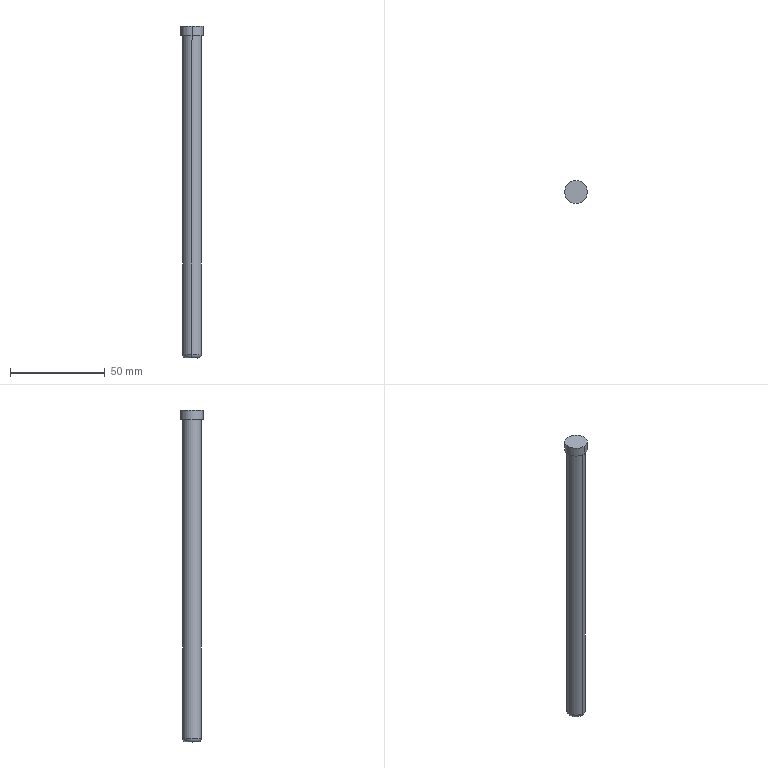Component | SolidWorks | 2SZT-2-003-5 | 1 solid | 9 faces | box 12 x 12 x 175 mm | volume 13893 mm3 | cylinder 4 | plane 3 | torus 2 | commonest cylinder face diameters 12 x2 10 x2
build123d program:
from build123d import *

# Parameters (mm, degrees)
SKETCH1_R           = 5
BOSS_EXTRUDE1_DEPTH = 170
SKETCH2_R           = 6
BOSS_EXTRUDE2_DEPTH = 5
FILLET1_R           = 2


with BuildPart() as part:
    # Sketch1 → Boss-Extrude1 (new body)
    with BuildSketch(Plane(origin=(0, 0, 0), x_dir=(1, 0, 0), z_dir=(0, 1, 0))):
        with Locations(Location((0, 0, 0), (0, 0, 270))):
            Circle(SKETCH1_R)
    extrude(amount=BOSS_EXTRUDE1_DEPTH)

    # Sketch2 → Boss-Extrude2 (add)
    with BuildSketch(Plane.XZ):
        with Locations(Location((0, 0, 0), (0, 0, 270))):
            Circle(SKETCH2_R)
    extrude(amount=BOSS_EXTRUDE2_DEPTH)

    # Fillet1
    fillet1_edges = [part.edges().sort_by_distance(p)[0] for p in [
        (0, 170, -5),
    ]]
    fillet(fillet1_edges, radius=FILLET1_R)


solid = part.part

# Placed as in the assembly
solid = solid.moved(Location((1050.266, 384.385, -180.948), (-90, 0, 0)))
STEP:
#1=COLOUR_RGB('',0.7922,0.8196,0.9333);
#2=FILL_AREA_STYLE_COLOUR('',#1);
#3=FILL_AREA_STYLE('',(#2));
#4=SURFACE_STYLE_FILL_AREA(#3);
#5=SURFACE_SIDE_STYLE('',(#4));
#6=SURFACE_STYLE_USAGE(.BOTH.,#5);
#7=PRESENTATION_STYLE_ASSIGNMENT((#6));
#8=CARTESIAN_POINT('',(41.349,14.936,-13.738));
#9=VERTEX_POINT('',#8);
#10=CARTESIAN_POINT('',(41.349,15.33,-13.738));
#11=VERTEX_POINT('',#10);
#12=CARTESIAN_POINT('',(41.349,15.133,-13.738));
#13=DIRECTION('',(0.00002551,0.,1.));
#14=DIRECTION('',(-0.00002551,1.,0.));
#15=AXIS2_PLACEMENT_3D('',#12,#13,#14);
#16=CIRCLE('',#15,0.1969);
#17=EDGE_CURVE('',#9,#11,#16,.T.);
#18=ORIENTED_EDGE('',*,*,#17,.F.);
#19=CARTESIAN_POINT('',(41.349,15.015,-13.817));
#20=VERTEX_POINT('',#19);
#21=CARTESIAN_POINT('',(41.349,15.015,-13.738));
#22=DIRECTION('',(1.,0.00002551,-0.00002551));
#23=DIRECTION('',(-0.00002551,1.,0.));
#24=AXIS2_PLACEMENT_3D('',#21,#22,#23);
#25=CIRCLE('',#24,0.07874);
#26=EDGE_CURVE('',#9,#20,#25,.T.);
#27=ORIENTED_EDGE('',*,*,#26,.T.);
#28=CARTESIAN_POINT('',(41.349,15.251,-13.817));
#29=VERTEX_POINT('',#28);
#30=CARTESIAN_POINT('',(41.349,15.133,-13.817));
#31=DIRECTION('',(-0.00002551,-0.,-1.));
#32=DIRECTION('',(-0.00002551,1.,0.));
#33=AXIS2_PLACEMENT_3D('',#30,#31,#32);
#34=CIRCLE('',#33,0.1181);
#35=EDGE_CURVE('',#29,#20,#34,.T.);
#36=ORIENTED_EDGE('',*,*,#35,.F.);
#37=CARTESIAN_POINT('',(41.349,15.251,-13.738));
#38=DIRECTION('',(-1.,-0.00002551,0.00002551));
#39=DIRECTION('',(0.00002551,-1.,0.));
#40=AXIS2_PLACEMENT_3D('',#37,#38,#39);
#41=CIRCLE('',#40,0.07874);
#42=EDGE_CURVE('',#11,#29,#41,.T.);
#43=ORIENTED_EDGE('',*,*,#42,.F.);
#44=EDGE_LOOP('',(#18,#27,#36,#43));
#45=FACE_OUTER_BOUND('',#44,.T.);
#46=CARTESIAN_POINT('',(41.349,15.133,-13.738));
#47=DIRECTION('',(-0.00002551,-0.,-1.));
#48=DIRECTION('',(-0.00002551,1.,0.));
#49=AXIS2_PLACEMENT_3D('',#46,#47,#48);
#50=TOROIDAL_SURFACE('',#49,0.1181,0.07874);
#51=ADVANCED_FACE('',(#45),#50,.T.);
#52=CARTESIAN_POINT('',(41.349,14.897,-6.927));
#53=VERTEX_POINT('',#52);
#54=CARTESIAN_POINT('',(41.349,15.369,-6.927));
#55=VERTEX_POINT('',#54);
#56=CARTESIAN_POINT('',(41.349,15.133,-6.927));
#57=DIRECTION('',(0.00002551,0.,1.));
#58=DIRECTION('',(0.00002551,-1.,-0.));
#59=AXIS2_PLACEMENT_3D('',#56,#57,#58);
#60=CIRCLE('',#59,0.2362);
#61=EDGE_CURVE('',#53,#55,#60,.T.);
#62=ORIENTED_EDGE('',*,*,#61,.F.);
#63=CARTESIAN_POINT('',(41.349,14.897,-7.124));
#64=VERTEX_POINT('',#63);
#65=CARTESIAN_POINT('',(41.349,14.897,-6.927));
#66=DIRECTION('',(-0.00002551,-0.,-1.));
#67=VECTOR('',#66,39.37);
#68=LINE('',#65,#67);
#69=EDGE_CURVE('',#53,#64,#68,.T.);
#70=ORIENTED_EDGE('',*,*,#69,.T.);
#71=CARTESIAN_POINT('',(41.349,15.369,-7.124));
#72=VERTEX_POINT('',#71);
#73=CARTESIAN_POINT('',(41.349,15.133,-7.124));
#74=DIRECTION('',(0.00002551,0.,1.));
#75=DIRECTION('',(0.00002551,-1.,-0.));
#76=AXIS2_PLACEMENT_3D('',#73,#74,#75);
#77=CIRCLE('',#76,0.2362);
#78=EDGE_CURVE('',#64,#72,#77,.T.);
#79=ORIENTED_EDGE('',*,*,#78,.T.);
#80=CARTESIAN_POINT('',(41.349,15.369,-6.927));
#81=DIRECTION('',(-0.00002551,-0.,-1.));
#82=VECTOR('',#81,39.37);
#83=LINE('',#80,#82);
#84=EDGE_CURVE('',#55,#72,#83,.T.);
#85=ORIENTED_EDGE('',*,*,#84,.F.);
#86=EDGE_LOOP('',(#62,#70,#79,#85));
#87=FACE_OUTER_BOUND('',#86,.T.);
#88=CARTESIAN_POINT('',(41.349,15.133,-6.927));
#89=DIRECTION('',(-0.00002551,-0.,-1.));
#90=DIRECTION('',(-0.00002551,1.,0.));
#91=AXIS2_PLACEMENT_3D('',#88,#89,#90);
#92=CYLINDRICAL_SURFACE('',#91,0.2362);
#93=ADVANCED_FACE('',(#87),#92,.T.);
#94=ORIENTED_EDGE('',*,*,#17,.T.);
#95=CARTESIAN_POINT('',(41.349,15.33,-7.124));
#96=VERTEX_POINT('',#95);
#97=CARTESIAN_POINT('',(41.349,15.33,-13.817));
#98=DIRECTION('',(0.00002551,0.,1.));
#99=VECTOR('',#98,39.37);
#100=LINE('',#97,#99);
#101=EDGE_CURVE('',#11,#96,#100,.T.);
#102=ORIENTED_EDGE('',*,*,#101,.T.);
#103=CARTESIAN_POINT('',(41.349,14.936,-7.124));
#104=VERTEX_POINT('',#103);
#105=CARTESIAN_POINT('',(41.349,15.133,-7.124));
#106=DIRECTION('',(0.00002551,0.,1.));
#107=DIRECTION('',(0.00002551,-1.,-0.));
#108=AXIS2_PLACEMENT_3D('',#105,#106,#107);
#109=CIRCLE('',#108,0.1969);
#110=EDGE_CURVE('',#104,#96,#109,.T.);
#111=ORIENTED_EDGE('',*,*,#110,.F.);
#112=CARTESIAN_POINT('',(41.349,14.936,-13.817));
#113=DIRECTION('',(0.00002551,0.,1.));
#114=VECTOR('',#113,39.37);
#115=LINE('',#112,#114);
#116=EDGE_CURVE('',#9,#104,#115,.T.);
#117=ORIENTED_EDGE('',*,*,#116,.F.);
#118=EDGE_LOOP('',(#94,#102,#111,#117));
#119=FACE_OUTER_BOUND('',#118,.T.);
#120=CARTESIAN_POINT('',(41.349,15.133,-13.817));
#121=DIRECTION('',(0.00002551,0.,1.));
#122=DIRECTION('',(0.00002551,-1.,-0.));
#123=AXIS2_PLACEMENT_3D('',#120,#121,#122);
#124=CYLINDRICAL_SURFACE('',#123,0.1969);
#125=ADVANCED_FACE('',(#119),#124,.T.);
#126=ORIENTED_EDGE('',*,*,#101,.F.);
#127=CARTESIAN_POINT('',(41.349,15.133,-13.738));
#128=DIRECTION('',(0.00002551,0.,1.));
#129=DIRECTION('',(-0.00002551,1.,0.));
#130=AXIS2_PLACEMENT_3D('',#127,#128,#129);
#131=CIRCLE('',#130,0.1969);
#132=EDGE_CURVE('',#11,#9,#131,.T.);
#133=ORIENTED_EDGE('',*,*,#132,.T.);
#134=ORIENTED_EDGE('',*,*,#116,.T.);
#135=CARTESIAN_POINT('',(41.349,15.133,-7.124));
#136=DIRECTION('',(0.00002551,0.,1.));
#137=DIRECTION('',(0.00002551,-1.,-0.));
#138=AXIS2_PLACEMENT_3D('',#135,#136,#137);
#139=CIRCLE('',#138,0.1969);
#140=EDGE_CURVE('',#96,#104,#139,.T.);
#141=ORIENTED_EDGE('',*,*,#140,.F.);
#142=EDGE_LOOP('',(#126,#133,#134,#141));
#143=FACE_OUTER_BOUND('',#142,.T.);
#144=CARTESIAN_POINT('',(41.349,15.133,-13.817));
#145=DIRECTION('',(0.00002551,0.,1.));
#146=DIRECTION('',(0.00002551,-1.,-0.));
#147=AXIS2_PLACEMENT_3D('',#144,#145,#146);
#148=CYLINDRICAL_SURFACE('',#147,0.1969);
#149=ADVANCED_FACE('',(#143),#148,.T.);
#150=ORIENTED_EDGE('',*,*,#35,.T.);
#151=CARTESIAN_POINT('',(41.349,15.133,-13.817));
#152=DIRECTION('',(-0.00002551,-0.,-1.));
#153=DIRECTION('',(-0.00002551,1.,0.));
#154=AXIS2_PLACEMENT_3D('',#151,#152,#153);
#155=CIRCLE('',#154,0.1181);
#156=EDGE_CURVE('',#20,#29,#155,.T.);
#157=ORIENTED_EDGE('',*,*,#156,.T.);
#158=EDGE_LOOP('',(#150,#157));
#159=FACE_OUTER_BOUND('',#158,.T.);
#160=CARTESIAN_POINT('',(41.349,15.133,-13.817));
#161=DIRECTION('',(-0.00002551,-0.,-1.));
#162=DIRECTION('',(-0.00002551,1.,0.));
#163=AXIS2_PLACEMENT_3D('',#160,#161,#162);
#164=PLANE('',#163);
#165=ADVANCED_FACE('',(#159),#164,.T.);
#166=CARTESIAN_POINT('',(41.349,15.133,-7.124));
#167=DIRECTION('',(0.00002551,0.,1.));
#168=DIRECTION('',(0.00002551,-1.,-0.));
#169=AXIS2_PLACEMENT_3D('',#166,#167,#168);
#170=CIRCLE('',#169,0.2362);
#171=EDGE_CURVE('',#72,#64,#170,.T.);
#172=ORIENTED_EDGE('',*,*,#171,.F.);
#173=ORIENTED_EDGE('',*,*,#78,.F.);
#174=EDGE_LOOP('',(#172,#173));
#175=FACE_OUTER_BOUND('',#174,.T.);
#176=ORIENTED_EDGE('',*,*,#110,.T.);
#177=ORIENTED_EDGE('',*,*,#140,.T.);
#178=EDGE_LOOP('',(#176,#177));
#179=FACE_BOUND('',#178,.T.);
#180=CARTESIAN_POINT('',(41.349,15.133,-7.124));
#181=DIRECTION('',(0.00002551,0.,1.));
#182=DIRECTION('',(0.00002551,-1.,-0.));
#183=AXIS2_PLACEMENT_3D('',#180,#181,#182);
#184=PLANE('',#183);
#185=ADVANCED_FACE('',(#175,#179),#184,.F.);
#186=ORIENTED_EDGE('',*,*,#69,.F.);
#187=CARTESIAN_POINT('',(41.349,15.133,-6.927));
#188=DIRECTION('',(0.00002551,0.,1.));
#189=DIRECTION('',(0.00002551,-1.,-0.));
#190=AXIS2_PLACEMENT_3D('',#187,#188,#189);
#191=CIRCLE('',#190,0.2362);
#192=EDGE_CURVE('',#55,#53,#191,.T.);
#193=ORIENTED_EDGE('',*,*,#192,.F.);
#194=ORIENTED_EDGE('',*,*,#84,.T.);
#195=ORIENTED_EDGE('',*,*,#171,.T.);
#196=EDGE_LOOP('',(#186,#193,#194,#195));
#197=FACE_OUTER_BOUND('',#196,.T.);
#198=CARTESIAN_POINT('',(41.349,15.133,-6.927));
#199=DIRECTION('',(-0.00002551,-0.,-1.));
#200=DIRECTION('',(-0.00002551,1.,0.));
#201=AXIS2_PLACEMENT_3D('',#198,#199,#200);
#202=CYLINDRICAL_SURFACE('',#201,0.2362);
#203=ADVANCED_FACE('',(#197),#202,.T.);
#204=ORIENTED_EDGE('',*,*,#192,.T.);
#205=ORIENTED_EDGE('',*,*,#61,.T.);
#206=EDGE_LOOP('',(#204,#205));
#207=FACE_OUTER_BOUND('',#206,.T.);
#208=CARTESIAN_POINT('',(41.349,15.133,-6.927));
#209=DIRECTION('',(0.00002551,0.,1.));
#210=DIRECTION('',(0.00002551,-1.,-0.));
#211=AXIS2_PLACEMENT_3D('',#208,#209,#210);
#212=PLANE('',#211);
#213=ADVANCED_FACE('',(#207),#212,.T.);
#214=ORIENTED_EDGE('',*,*,#26,.F.);
#215=ORIENTED_EDGE('',*,*,#132,.F.);
#216=ORIENTED_EDGE('',*,*,#42,.T.);
#217=ORIENTED_EDGE('',*,*,#156,.F.);
#218=EDGE_LOOP('',(#214,#215,#216,#217));
#219=FACE_OUTER_BOUND('',#218,.T.);
#220=CARTESIAN_POINT('',(41.349,15.133,-13.738));
#221=DIRECTION('',(-0.00002551,-0.,-1.));
#222=DIRECTION('',(-0.00002551,1.,0.));
#223=AXIS2_PLACEMENT_3D('',#220,#221,#222);
#224=TOROIDAL_SURFACE('',#223,0.1181,0.07874);
#225=ADVANCED_FACE('',(#219),#224,.T.);
#226=CLOSED_SHELL('',(#51,#93,#125,#149,#165,#185,#203,#213,#225));
#227=MANIFOLD_SOLID_BREP('',#226);
#228=STYLED_ITEM('',(#7),#227);
#229=PRESENTATION_LAYER_ASSIGNMENT('','',(#228));
#230=CARTESIAN_POINT('',(0.,0.,0.));
#231=DIRECTION('',(0.,0.,1.));
#232=DIRECTION('',(1.,0.,0.));
#233=AXIS2_PLACEMENT_3D('',#230,#231,#232);
#234=(LENGTH_UNIT()NAMED_UNIT(*)SI_UNIT($,.METRE.));
#235=LENGTH_MEASURE_WITH_UNIT(LENGTH_MEASURE(0.0254),#234);
#236=DIMENSIONAL_EXPONENTS(1.,0.,0.,0.,0.,0.,0.);
#237=(CONVERSION_BASED_UNIT('',#235)LENGTH_UNIT()NAMED_UNIT(#236));
#238=UNCERTAINTY_MEASURE_WITH_UNIT(LENGTH_MEASURE(0.00001),#237,'','');
#239=(NAMED_UNIT(*)PLANE_ANGLE_UNIT()SI_UNIT($,.RADIAN.));
#240=(NAMED_UNIT(*)SI_UNIT($,.STERADIAN.)SOLID_ANGLE_UNIT());
#241=(GEOMETRIC_REPRESENTATION_CONTEXT(3)GLOBAL_UNCERTAINTY_ASSIGNED_CONTEXT((#238))GLOBAL_UNIT_ASSIGNED_CONTEXT((#237,#239,#240))REPRESENTATION_CONTEXT('',''));
#242=ADVANCED_BREP_SHAPE_REPRESENTATION('',(#227,#233),#241);
#243=(LENGTH_UNIT()NAMED_UNIT(*)SI_UNIT($,.METRE.));
#244=LENGTH_MEASURE_WITH_UNIT(LENGTH_MEASURE(0.0254),#243);
#245=DIMENSIONAL_EXPONENTS(1.,0.,0.,0.,0.,0.,0.);
#246=(CONVERSION_BASED_UNIT('',#244)LENGTH_UNIT()NAMED_UNIT(#245));
#247=UNCERTAINTY_MEASURE_WITH_UNIT(LENGTH_MEASURE(0.00001),#246,'','');
#248=(NAMED_UNIT(*)PLANE_ANGLE_UNIT()SI_UNIT($,.RADIAN.));
#249=(NAMED_UNIT(*)SI_UNIT($,.STERADIAN.)SOLID_ANGLE_UNIT());
#250=(GEOMETRIC_REPRESENTATION_CONTEXT(3)GLOBAL_UNCERTAINTY_ASSIGNED_CONTEXT((#247))GLOBAL_UNIT_ASSIGNED_CONTEXT((#246,#248,#249))REPRESENTATION_CONTEXT('',''));
#251=MECHANICAL_DESIGN_GEOMETRIC_PRESENTATION_REPRESENTATION('',(#228),#250);